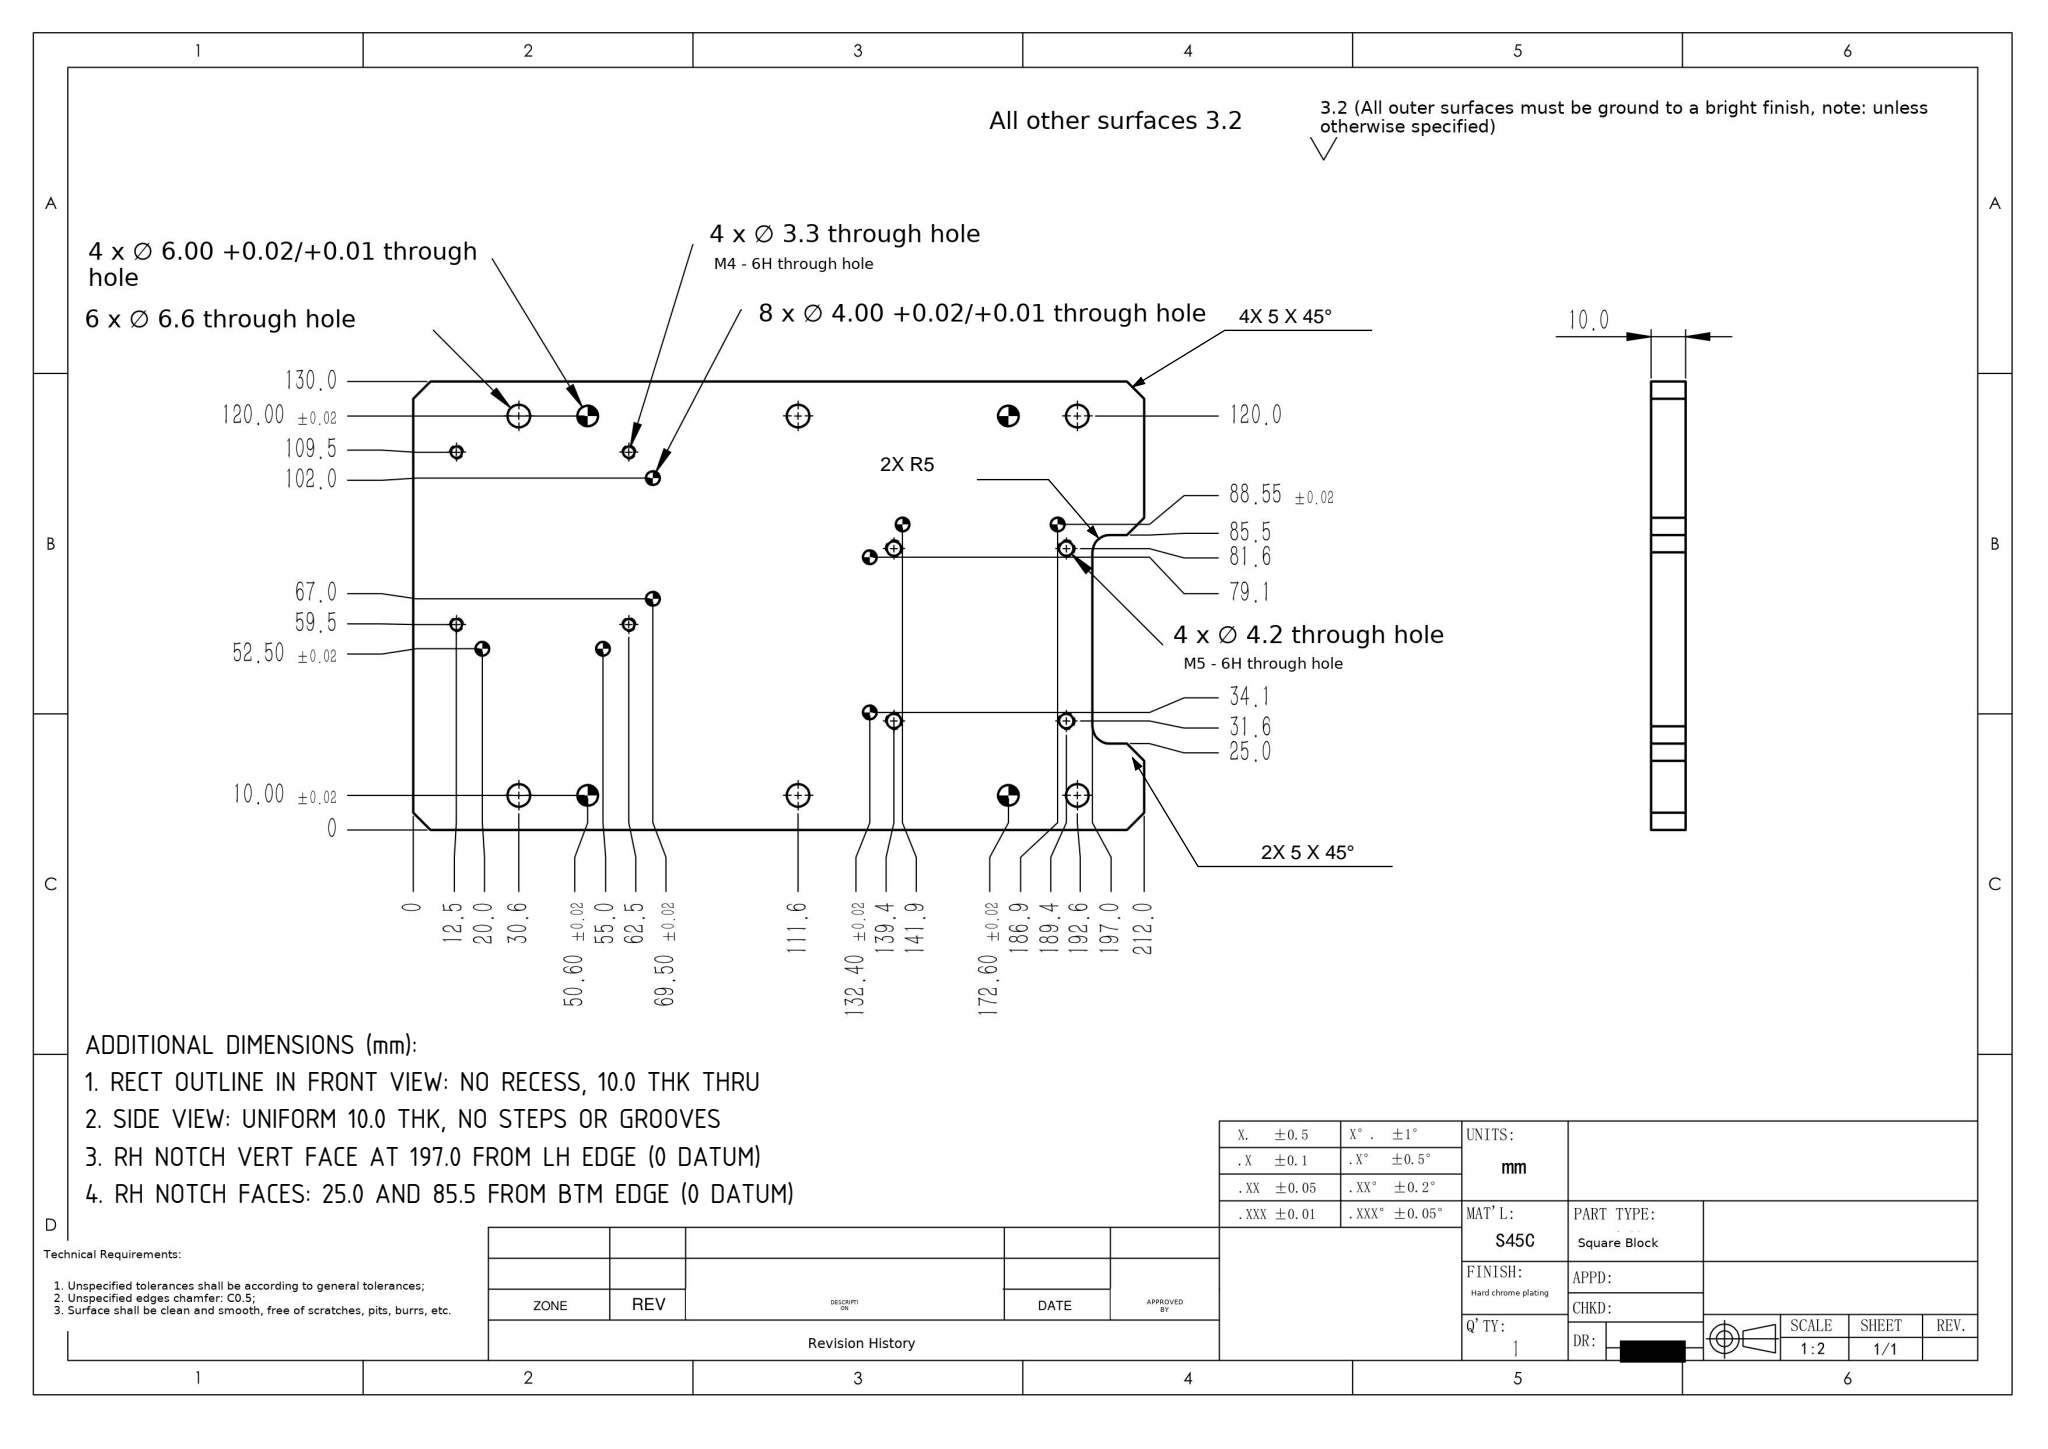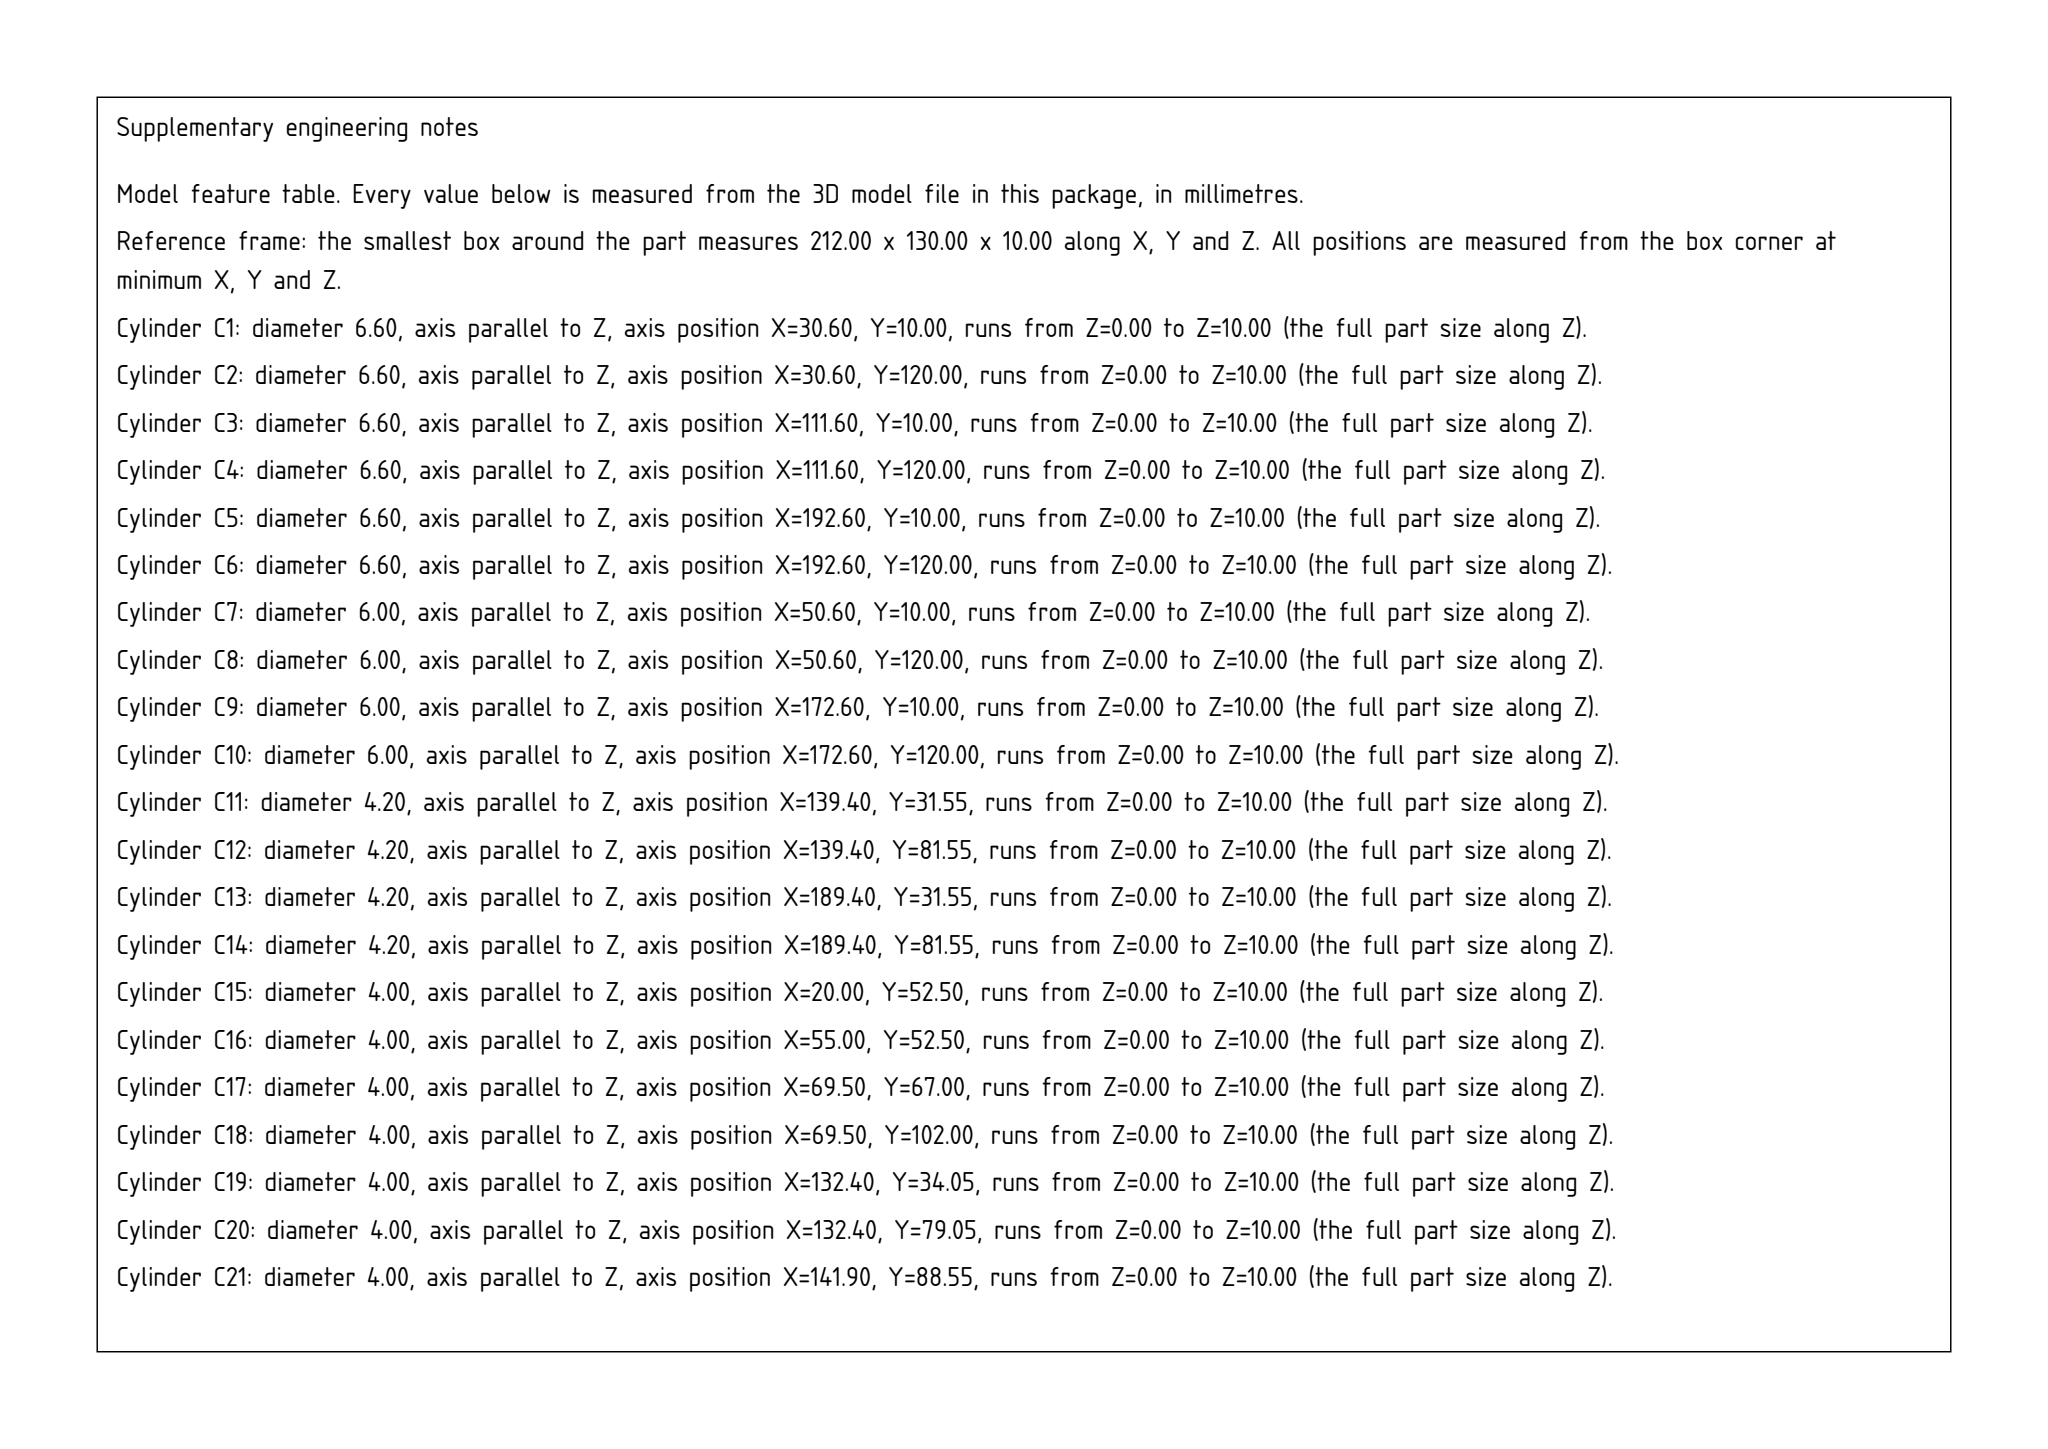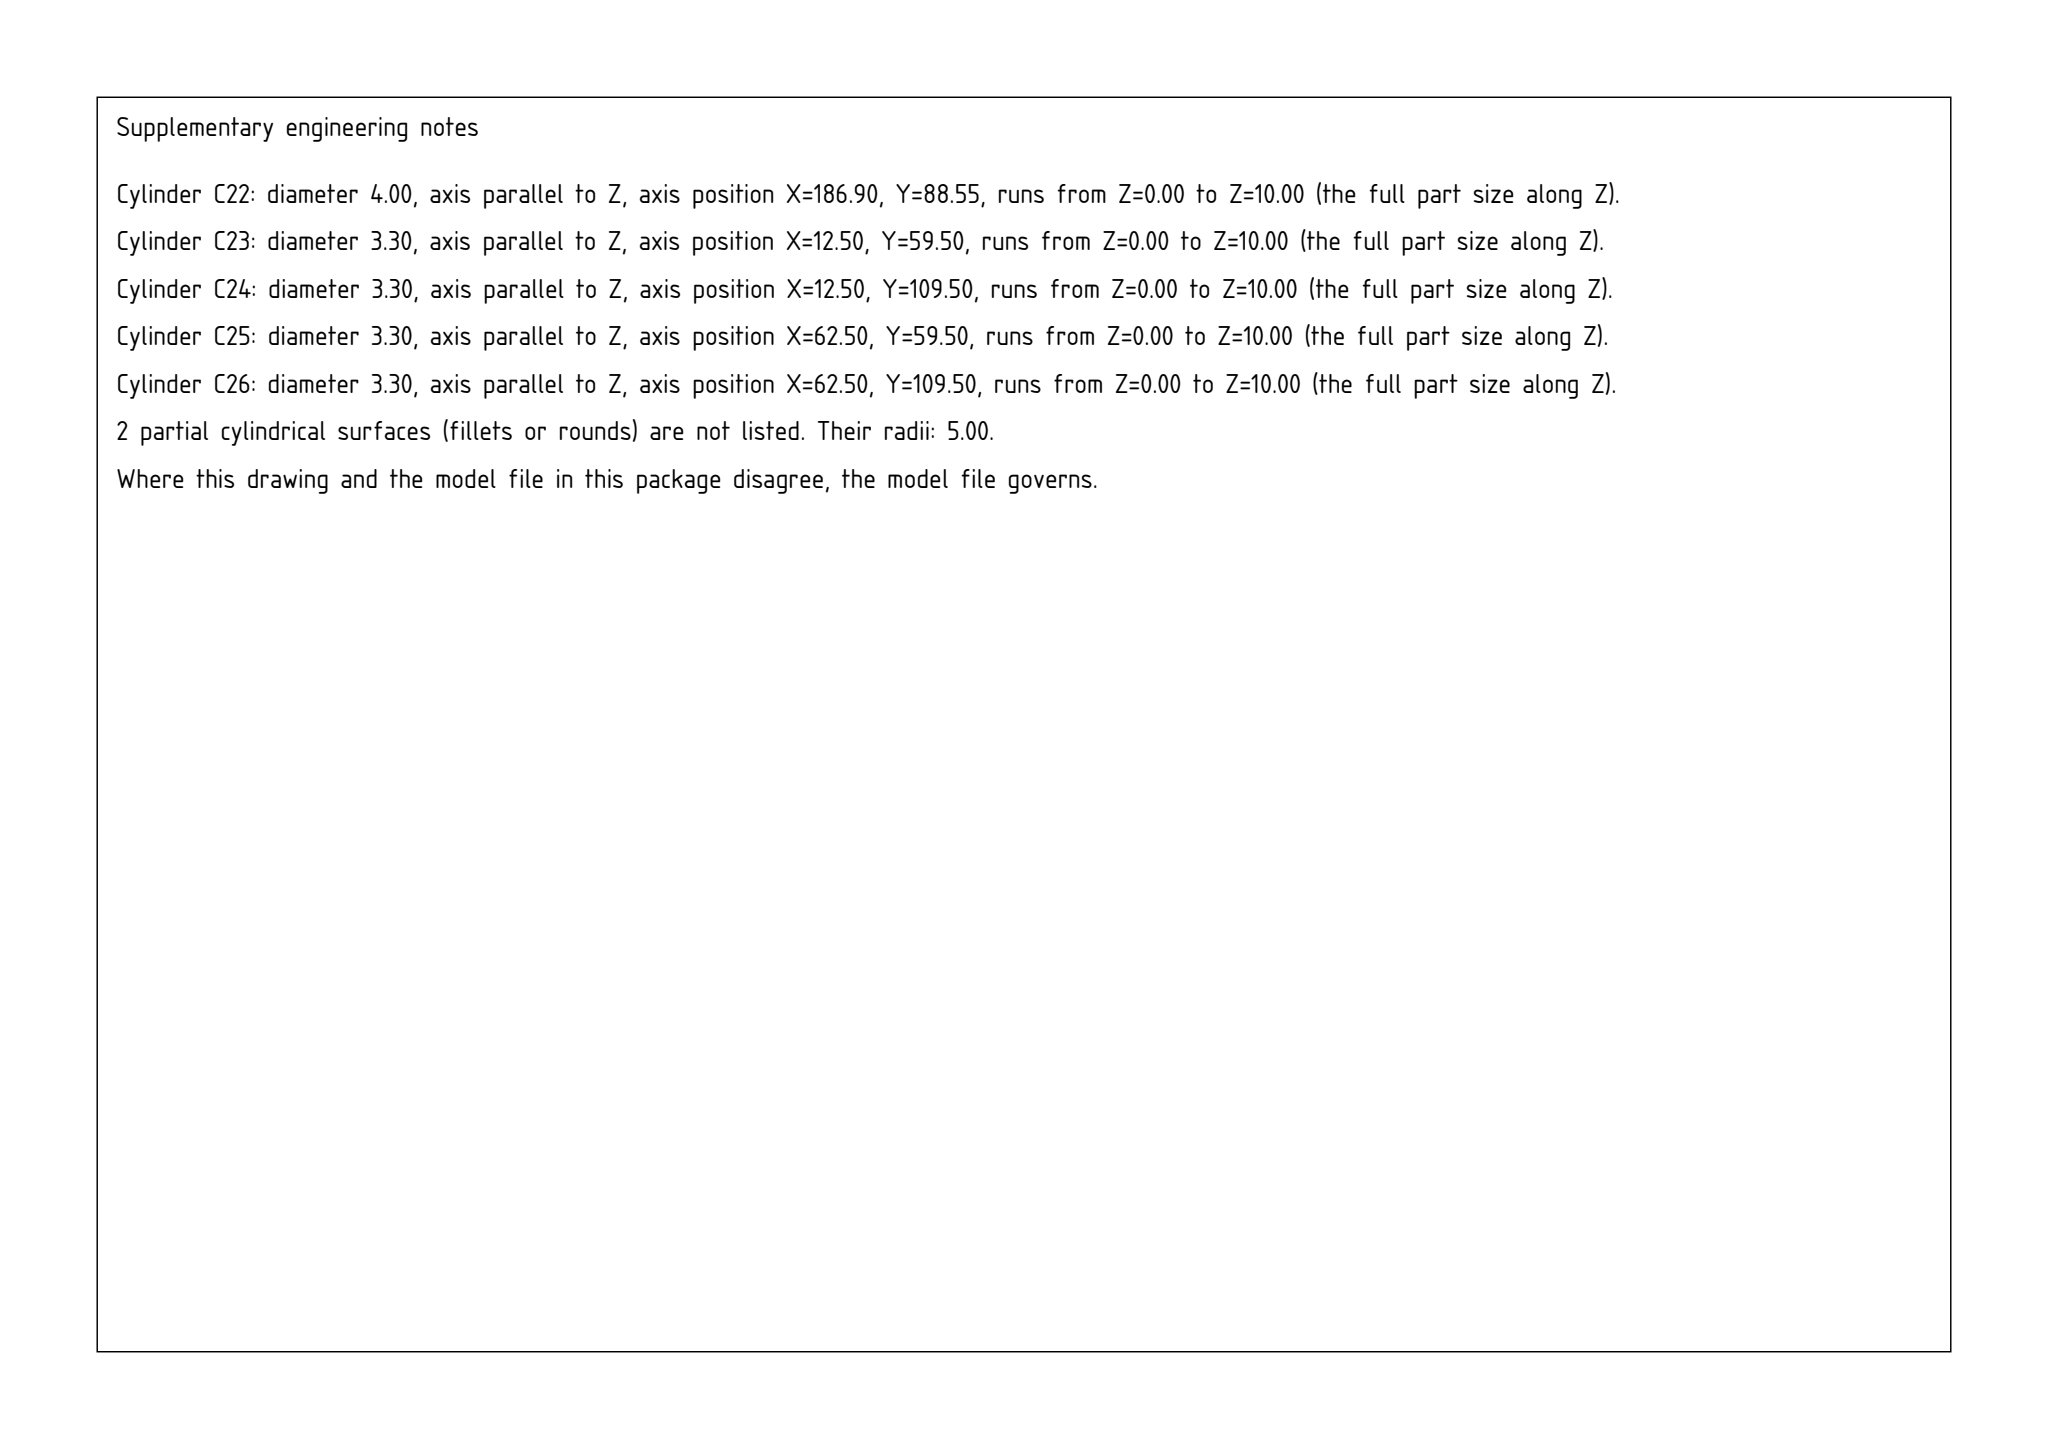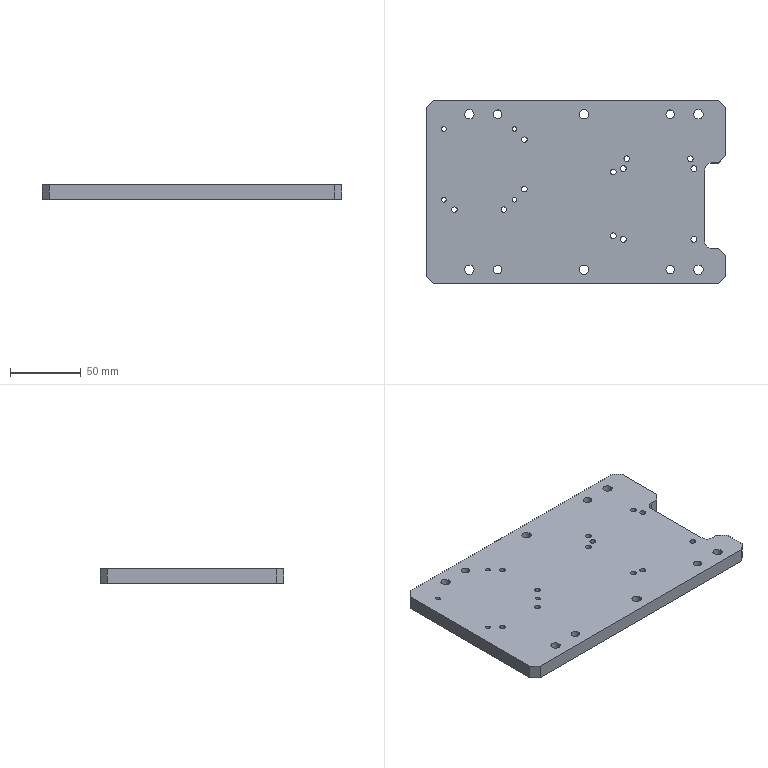Part | SolidWorks | mm | 1 solid | 70 faces | box 212 x 130 x 10 mm | volume 260797 mm3 | cylinder 54 | plane 16 | commonest cylinder face diameters 4 x16 6.6 x12 6 x8 4.2 x8 3.3 x8 10 x2
build123d program:
from build123d import *

# Parameters (mm, degrees)
SKETCH1_W                 = 212
SKETCH1_H                 = 130
BOSS_EXTRUDE1_DEPTH       = 10
SKETCH2_W                 = 15
SKETCH2_H                 = 60.5
CUT_EXTRUDE1_DEPTH        = 125.744
M4_TAPPED_HOLE1_D         = 3.3
M5_TAPPED_HOLE1_D         = 4.2
SIZE_MM_DOWEL_PIN_HOLE1_D = 4
SIZE_MM_DOWEL_PIN_HOLE2_D = 6
M6_CLEARANCE_HOLE1_D      = 6.6
CHAMFER1_SIZE             = 5
FILLET1_R                 = 5


with BuildPart() as part:
    # Sketch1 → Boss-Extrude1 (new body)
    with BuildSketch(Plane.XY):
        Rectangle(SKETCH1_W, SKETCH1_H)
    extrude(amount=BOSS_EXTRUDE1_DEPTH)

    # Sketch2 → Cut-Extrude1 (cut, through all)
    with BuildSketch(Plane.XY.offset(10)):
        with Locations((98.5, -9.75)):
            Rectangle(SKETCH2_W, SKETCH2_H)
    extrude(amount=-CUT_EXTRUDE1_DEPTH, mode=Mode.SUBTRACT)

    # M4 Tapped Hole1 (through all)
    with Locations(Plane(origin=(0, 0, 0), x_dir=(-1, 0, 0), z_dir=(0, 0, -1))):
        with Locations((93.5, 44.5), (43.5, 44.5), (93.5, -5.5), (43.5, -5.5)):
            Hole(M4_TAPPED_HOLE1_D / 2)

    # M5 Tapped Hole1 (through all)
    with Locations(Plane.XY.offset(10)):
        with Locations((83.4, 16.55), (83.4, -33.45), (33.4, -33.45), (33.4, 16.55)):
            Hole(M5_TAPPED_HOLE1_D / 2)

    # Size mm Dowel Pin Hole1 (through all)
    with Locations(Plane.XY.offset(10)):
        with Locations((-86, -12.5), (-51, -12.5), (-36.5, 2), (-36.5, 37), (35.9, 23.55), (80.9, 23.55), (26.4, 14.05), (26.4, -30.95)):
            Hole(SIZE_MM_DOWEL_PIN_HOLE1_D / 2)

    # Size mm Dowel Pin Hole2 (through all)
    with Locations(Plane.XY.offset(10)):
        with Locations((-55.4, -55), (66.6, -55), (66.6, 55), (-55.4, 55)):
            Hole(SIZE_MM_DOWEL_PIN_HOLE2_D / 2)

    # M6 Clearance Hole1 (through all)
    with Locations(Plane.XY.offset(10)):
        with Locations((-75.4, -55), (86.6, -55), (86.6, 55), (-75.4, 55), (5.6, -55), (5.6, 55)):
            Hole(M6_CLEARANCE_HOLE1_D / 2)

    # Chamfer1
    chamfer1_edges = [part.edges().sort_by_distance(p)[0] for p in [
        (106, 20.5, 5),
        (106, -40, 5),
        (106, -65, 5),
        (-106, -65, 5),
        (-106, 65, 5),
        (106, 65, 5),
    ]]
    chamfer(chamfer1_edges, length=CHAMFER1_SIZE)

    # Fillet1
    fillet1_edges = [part.edges().sort_by_distance(p)[0] for p in [
        (91, -40, 5),
        (91, 20.5, 5),
    ]]
    fillet(fillet1_edges, radius=FILLET1_R)


solid = part.part